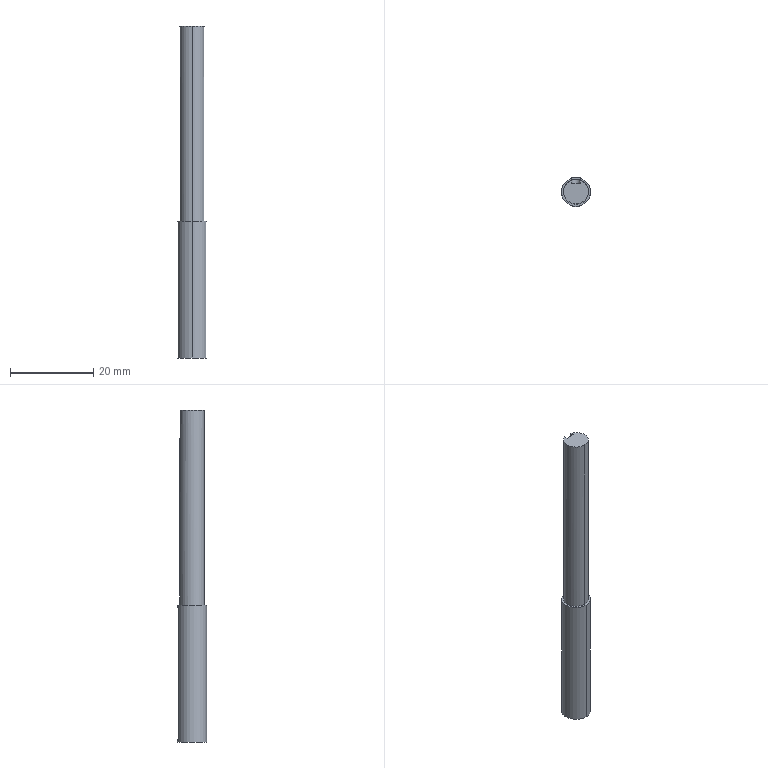Component | SolidWorks | DriveAxis-1 | 1 solid | 16 faces | box 7 x 7 x 80 mm | volume 2512 mm3 | plane 9 | cylinder 7 | commonest cylinder face diameters 6 x2 7 x2 2.5 x2 2 x1
build123d program:
from build123d import *

# Parameters (mm, degrees)
SKETCH1_R           = 3.5
BOSS_EXTRUDE1_DEPTH = 33
SKETCH2_R           = 3
BOSS_EXTRUDE2_DEPTH = 47
CUT_EXTRUDE1_DEPTH  = 1
CUT_EXTRUDE2_DEPTH  = 1


with BuildPart() as part:
    # Sketch1 → Boss-Extrude1 (new body)
    with BuildSketch(Plane(origin=(0, 0, 0), x_dir=(1, 0, 0), z_dir=(0, 1, 0))):
        with Locations(Location((0, 0, 0), (0, 0, 270))):
            Circle(SKETCH1_R)
    extrude(amount=BOSS_EXTRUDE1_DEPTH)

    # Sketch2 → Boss-Extrude2 (add)
    with BuildSketch(Plane(origin=(0, 33, 0), x_dir=(1, 0, 0), z_dir=(0, 1, 0))):
        with Locations(Location((0, 0, 0), (0, 0, 270))):
            Circle(SKETCH2_R)
    extrude(amount=BOSS_EXTRUDE2_DEPTH)

    # Sketch3 → Cut-Extrude1 (cut)
    with BuildSketch(Plane(origin=(0, 0, -3.5), x_dir=(-1, 0, 0), z_dir=(0, 0, -1))):
        with BuildLine():
            Line((1.25, 31.498), (1.25, 1.498))
            ThreePointArc((1.25, 1.498), (0, 0.2475), (-1.25, 1.498))
            Line((-1.25, 1.498), (-1.25, 31.498))
            ThreePointArc((-1.25, 31.498), (0, 32.748), (1.25, 31.498))
        make_face()
    extrude(amount=-CUT_EXTRUDE1_DEPTH, mode=Mode.SUBTRACT)

    # Sketch4 → Cut-Extrude2 (cut)
    with BuildSketch(Plane(origin=(0, 0, -3), x_dir=(-1, 0, 0), z_dir=(0, 0, -1))):
        with BuildLine():
            Line((1, 80), (1, 74))
            ThreePointArc((1, 74), (0, 73), (-1, 74))
            Line((-1, 74), (-1, 80))
            ThreePointArc((-1, 80), (0, 81), (1, 80))
        make_face()
    extrude(amount=-CUT_EXTRUDE2_DEPTH, mode=Mode.SUBTRACT)


solid = part.part

# Placed as in the assembly
solid = solid.moved(Location((48.507, -64.609, -275), (90, 0, 0)))
STEP:
#1=COLOUR_RGB('',0.7922,0.8196,0.9333);
#2=FILL_AREA_STYLE_COLOUR('',#1);
#3=FILL_AREA_STYLE('',(#2));
#4=SURFACE_STYLE_FILL_AREA(#3);
#5=SURFACE_SIDE_STYLE('',(#4));
#6=SURFACE_STYLE_USAGE(.BOTH.,#5);
#7=PRESENTATION_STYLE_ASSIGNMENT((#6));
#8=CARTESIAN_POINT('',(1.91,-2.662,-7.677));
#9=VERTEX_POINT('',#8);
#10=CARTESIAN_POINT('',(1.949,-2.432,-7.677));
#11=VERTEX_POINT('',#10);
#12=CARTESIAN_POINT('',(1.91,-2.544,-7.677));
#13=DIRECTION('',(0.,0.,1.));
#14=DIRECTION('',(0.,-1.,0.));
#15=AXIS2_PLACEMENT_3D('',#12,#13,#14);
#16=CIRCLE('',#15,0.1181);
#17=EDGE_CURVE('',#9,#11,#16,.T.);
#18=ORIENTED_EDGE('',*,*,#17,.F.);
#19=CARTESIAN_POINT('',(1.91,-2.662,-9.528));
#20=VERTEX_POINT('',#19);
#21=CARTESIAN_POINT('',(1.91,-2.662,-7.677));
#22=DIRECTION('',(0.,0.,-1.));
#23=VECTOR('',#22,39.37);
#24=LINE('',#21,#23);
#25=EDGE_CURVE('',#9,#20,#24,.T.);
#26=ORIENTED_EDGE('',*,*,#25,.T.);
#27=CARTESIAN_POINT('',(1.91,-2.426,-9.528));
#28=VERTEX_POINT('',#27);
#29=CARTESIAN_POINT('',(1.91,-2.544,-9.528));
#30=DIRECTION('',(0.,0.,1.));
#31=DIRECTION('',(0.,-1.,0.));
#32=AXIS2_PLACEMENT_3D('',#29,#30,#31);
#33=CIRCLE('',#32,0.1181);
#34=EDGE_CURVE('',#20,#28,#33,.T.);
#35=ORIENTED_EDGE('',*,*,#34,.T.);
#36=CARTESIAN_POINT('',(1.91,-2.426,-7.953));
#37=VERTEX_POINT('',#36);
#38=CARTESIAN_POINT('',(1.91,-2.426,-7.677));
#39=DIRECTION('',(0.,0.,-1.));
#40=VECTOR('',#39,39.37);
#41=LINE('',#38,#40);
#42=EDGE_CURVE('',#37,#28,#41,.T.);
#43=ORIENTED_EDGE('',*,*,#42,.F.);
#44=CARTESIAN_POINT('',(1.949,-2.432,-7.913));
#45=VERTEX_POINT('',#44);
#46=CARTESIAN_POINT('',(1.91,-2.426,-7.953));
#47=CARTESIAN_POINT('',(1.915,-2.426,-7.953));
#48=CARTESIAN_POINT('',(1.92,-2.426,-7.952));
#49=CARTESIAN_POINT('',(1.93,-2.427,-7.948));
#50=CARTESIAN_POINT('',(1.934,-2.428,-7.945));
#51=CARTESIAN_POINT('',(1.941,-2.43,-7.938));
#52=CARTESIAN_POINT('',(1.944,-2.431,-7.933));
#53=CARTESIAN_POINT('',(1.948,-2.432,-7.924));
#54=CARTESIAN_POINT('',(1.949,-2.432,-7.919));
#55=CARTESIAN_POINT('',(1.949,-2.432,-7.913));
#56=B_SPLINE_CURVE_WITH_KNOTS('',3,(#46,#47,#48,#49,#50,#51,#52,#53,#54,#55),.UNSPECIFIED.,.F.,.F.,(4,2,2,2,4),(0.001575,0.001968,0.002361,0.002755,0.003148),.UNSPECIFIED.);
#57=EDGE_CURVE('',#37,#45,#56,.T.);
#58=ORIENTED_EDGE('',*,*,#57,.T.);
#59=CARTESIAN_POINT('',(1.949,-2.432,-7.677));
#60=DIRECTION('',(0.,0.,1.));
#61=VECTOR('',#60,39.37);
#62=LINE('',#59,#61);
#63=EDGE_CURVE('',#45,#11,#62,.T.);
#64=ORIENTED_EDGE('',*,*,#63,.T.);
#65=EDGE_LOOP('',(#18,#26,#35,#43,#58,#64));
#66=FACE_OUTER_BOUND('',#65,.T.);
#67=CARTESIAN_POINT('',(1.91,-2.544,-7.677));
#68=DIRECTION('',(0.,0.,-1.));
#69=DIRECTION('',(0.,1.,0.));
#70=AXIS2_PLACEMENT_3D('',#67,#68,#69);
#71=CYLINDRICAL_SURFACE('',#70,0.1181);
#72=ADVANCED_FACE('',(#66),#71,.T.);
#73=CARTESIAN_POINT('',(1.91,-2.681,-9.528));
#74=VERTEX_POINT('',#73);
#75=CARTESIAN_POINT('',(1.91,-2.406,-9.528));
#76=VERTEX_POINT('',#75);
#77=CARTESIAN_POINT('',(1.91,-2.544,-9.528));
#78=DIRECTION('',(0.,0.,1.));
#79=DIRECTION('',(0.,-1.,0.));
#80=AXIS2_PLACEMENT_3D('',#77,#78,#79);
#81=CIRCLE('',#80,0.1378);
#82=EDGE_CURVE('',#74,#76,#81,.T.);
#83=ORIENTED_EDGE('',*,*,#82,.F.);
#84=CARTESIAN_POINT('',(1.91,-2.681,-10.827));
#85=VERTEX_POINT('',#84);
#86=CARTESIAN_POINT('',(1.91,-2.681,-9.528));
#87=DIRECTION('',(0.,0.,-1.));
#88=VECTOR('',#87,39.37);
#89=LINE('',#86,#88);
#90=EDGE_CURVE('',#74,#85,#89,.T.);
#91=ORIENTED_EDGE('',*,*,#90,.T.);
#92=CARTESIAN_POINT('',(1.91,-2.406,-10.827));
#93=VERTEX_POINT('',#92);
#94=CARTESIAN_POINT('',(1.91,-2.544,-10.827));
#95=DIRECTION('',(0.,0.,1.));
#96=DIRECTION('',(0.,-1.,0.));
#97=AXIS2_PLACEMENT_3D('',#94,#95,#96);
#98=CIRCLE('',#97,0.1378);
#99=EDGE_CURVE('',#85,#93,#98,.T.);
#100=ORIENTED_EDGE('',*,*,#99,.T.);
#101=CARTESIAN_POINT('',(1.91,-2.406,-10.817));
#102=VERTEX_POINT('',#101);
#103=CARTESIAN_POINT('',(1.91,-2.406,-9.528));
#104=DIRECTION('',(0.,0.,-1.));
#105=VECTOR('',#104,39.37);
#106=LINE('',#103,#105);
#107=EDGE_CURVE('',#102,#93,#106,.T.);
#108=ORIENTED_EDGE('',*,*,#107,.F.);
#109=CARTESIAN_POINT('',(1.959,-2.415,-10.768));
#110=VERTEX_POINT('',#109);
#111=CARTESIAN_POINT('',(1.91,-2.406,-10.817));
#112=CARTESIAN_POINT('',(1.913,-2.406,-10.817));
#113=CARTESIAN_POINT('',(1.916,-2.406,-10.817));
#114=CARTESIAN_POINT('',(1.923,-2.406,-10.815));
#115=CARTESIAN_POINT('',(1.926,-2.407,-10.814));
#116=CARTESIAN_POINT('',(1.935,-2.408,-10.811));
#117=CARTESIAN_POINT('',(1.94,-2.409,-10.807));
#118=CARTESIAN_POINT('',(1.947,-2.411,-10.8));
#119=CARTESIAN_POINT('',(1.949,-2.411,-10.798));
#120=CARTESIAN_POINT('',(1.952,-2.413,-10.793));
#121=CARTESIAN_POINT('',(1.954,-2.413,-10.79));
#122=CARTESIAN_POINT('',(1.958,-2.414,-10.781));
#123=CARTESIAN_POINT('',(1.959,-2.415,-10.774));
#124=CARTESIAN_POINT('',(1.959,-2.415,-10.768));
#125=B_SPLINE_CURVE_WITH_KNOTS('',3,(#111,#112,#113,#114,#115,#116,#117,#118,#119,#120,#121,#122,#123,#124),.UNSPECIFIED.,.F.,.F.,(4,2,2,2,2,2,4),(0.001971,0.002217,0.002463,0.002955,0.003201,0.003447,0.003939),.UNSPECIFIED.);
#126=EDGE_CURVE('',#102,#110,#125,.T.);
#127=ORIENTED_EDGE('',*,*,#126,.T.);
#128=CARTESIAN_POINT('',(1.959,-2.415,-9.587));
#129=VERTEX_POINT('',#128);
#130=CARTESIAN_POINT('',(1.959,-2.415,-9.528));
#131=DIRECTION('',(0.,0.,1.));
#132=VECTOR('',#131,39.37);
#133=LINE('',#130,#132);
#134=EDGE_CURVE('',#110,#129,#133,.T.);
#135=ORIENTED_EDGE('',*,*,#134,.T.);
#136=CARTESIAN_POINT('',(1.91,-2.406,-9.537));
#137=VERTEX_POINT('',#136);
#138=CARTESIAN_POINT('',(1.959,-2.415,-9.587));
#139=CARTESIAN_POINT('',(1.959,-2.415,-9.58));
#140=CARTESIAN_POINT('',(1.958,-2.414,-9.574));
#141=CARTESIAN_POINT('',(1.953,-2.413,-9.562));
#142=CARTESIAN_POINT('',(1.949,-2.411,-9.556));
#143=CARTESIAN_POINT('',(1.94,-2.409,-9.547));
#144=CARTESIAN_POINT('',(1.935,-2.408,-9.544));
#145=CARTESIAN_POINT('',(1.923,-2.406,-9.539));
#146=CARTESIAN_POINT('',(1.916,-2.406,-9.537));
#147=CARTESIAN_POINT('',(1.91,-2.406,-9.537));
#148=B_SPLINE_CURVE_WITH_KNOTS('',3,(#138,#139,#140,#141,#142,#143,#144,#145,#146,#147),.UNSPECIFIED.,.F.,.F.,(4,2,2,2,4),(0.,0.0004927,0.0009855,0.001478,0.001971),.UNSPECIFIED.);
#149=EDGE_CURVE('',#129,#137,#148,.T.);
#150=ORIENTED_EDGE('',*,*,#149,.T.);
#151=CARTESIAN_POINT('',(1.91,-2.406,-9.528));
#152=DIRECTION('',(0.,0.,-1.));
#153=VECTOR('',#152,39.37);
#154=LINE('',#151,#153);
#155=EDGE_CURVE('',#76,#137,#154,.T.);
#156=ORIENTED_EDGE('',*,*,#155,.F.);
#157=EDGE_LOOP('',(#83,#91,#100,#108,#127,#135,#150,#156));
#158=FACE_OUTER_BOUND('',#157,.T.);
#159=CARTESIAN_POINT('',(1.91,-2.544,-9.528));
#160=DIRECTION('',(0.,0.,-1.));
#161=DIRECTION('',(0.,1.,0.));
#162=AXIS2_PLACEMENT_3D('',#159,#160,#161);
#163=CYLINDRICAL_SURFACE('',#162,0.1378);
#164=ADVANCED_FACE('',(#158),#163,.T.);
#165=ORIENTED_EDGE('',*,*,#90,.F.);
#166=CARTESIAN_POINT('',(1.91,-2.544,-9.528));
#167=DIRECTION('',(0.,0.,1.));
#168=DIRECTION('',(0.,-1.,0.));
#169=AXIS2_PLACEMENT_3D('',#166,#167,#168);
#170=CIRCLE('',#169,0.1378);
#171=EDGE_CURVE('',#76,#74,#170,.T.);
#172=ORIENTED_EDGE('',*,*,#171,.F.);
#173=ORIENTED_EDGE('',*,*,#155,.T.);
#174=CARTESIAN_POINT('',(1.861,-2.415,-9.587));
#175=VERTEX_POINT('',#174);
#176=CARTESIAN_POINT('',(1.91,-2.406,-9.537));
#177=CARTESIAN_POINT('',(1.906,-2.406,-9.537));
#178=CARTESIAN_POINT('',(1.903,-2.406,-9.538));
#179=CARTESIAN_POINT('',(1.897,-2.406,-9.539));
#180=CARTESIAN_POINT('',(1.894,-2.407,-9.54));
#181=CARTESIAN_POINT('',(1.885,-2.408,-9.544));
#182=CARTESIAN_POINT('',(1.879,-2.409,-9.547));
#183=CARTESIAN_POINT('',(1.873,-2.411,-9.554));
#184=CARTESIAN_POINT('',(1.871,-2.411,-9.557));
#185=CARTESIAN_POINT('',(1.867,-2.413,-9.562));
#186=CARTESIAN_POINT('',(1.866,-2.413,-9.565));
#187=CARTESIAN_POINT('',(1.862,-2.414,-9.574));
#188=CARTESIAN_POINT('',(1.861,-2.415,-9.58));
#189=CARTESIAN_POINT('',(1.861,-2.415,-9.587));
#190=B_SPLINE_CURVE_WITH_KNOTS('',3,(#176,#177,#178,#179,#180,#181,#182,#183,#184,#185,#186,#187,#188,#189),.UNSPECIFIED.,.F.,.F.,(4,2,2,2,2,2,4),(0.001971,0.002217,0.002463,0.002955,0.003201,0.003447,0.003939),.UNSPECIFIED.);
#191=EDGE_CURVE('',#137,#175,#190,.T.);
#192=ORIENTED_EDGE('',*,*,#191,.T.);
#193=CARTESIAN_POINT('',(1.861,-2.415,-10.768));
#194=VERTEX_POINT('',#193);
#195=CARTESIAN_POINT('',(1.861,-2.415,-9.528));
#196=DIRECTION('',(0.,0.,-1.));
#197=VECTOR('',#196,39.37);
#198=LINE('',#195,#197);
#199=EDGE_CURVE('',#175,#194,#198,.T.);
#200=ORIENTED_EDGE('',*,*,#199,.T.);
#201=CARTESIAN_POINT('',(1.861,-2.415,-10.768));
#202=CARTESIAN_POINT('',(1.861,-2.415,-10.774));
#203=CARTESIAN_POINT('',(1.862,-2.414,-10.781));
#204=CARTESIAN_POINT('',(1.867,-2.413,-10.793));
#205=CARTESIAN_POINT('',(1.87,-2.411,-10.798));
#206=CARTESIAN_POINT('',(1.879,-2.409,-10.807));
#207=CARTESIAN_POINT('',(1.885,-2.408,-10.811));
#208=CARTESIAN_POINT('',(1.897,-2.406,-10.816));
#209=CARTESIAN_POINT('',(1.903,-2.406,-10.817));
#210=CARTESIAN_POINT('',(1.91,-2.406,-10.817));
#211=B_SPLINE_CURVE_WITH_KNOTS('',3,(#201,#202,#203,#204,#205,#206,#207,#208,#209,#210),.UNSPECIFIED.,.F.,.F.,(4,2,2,2,4),(0.,0.0004927,0.0009855,0.001478,0.001971),.UNSPECIFIED.);
#212=EDGE_CURVE('',#194,#102,#211,.T.);
#213=ORIENTED_EDGE('',*,*,#212,.T.);
#214=ORIENTED_EDGE('',*,*,#107,.T.);
#215=CARTESIAN_POINT('',(1.91,-2.544,-10.827));
#216=DIRECTION('',(0.,0.,1.));
#217=DIRECTION('',(0.,-1.,0.));
#218=AXIS2_PLACEMENT_3D('',#215,#216,#217);
#219=CIRCLE('',#218,0.1378);
#220=EDGE_CURVE('',#93,#85,#219,.T.);
#221=ORIENTED_EDGE('',*,*,#220,.T.);
#222=EDGE_LOOP('',(#165,#172,#173,#192,#200,#213,#214,#221));
#223=FACE_OUTER_BOUND('',#222,.T.);
#224=CARTESIAN_POINT('',(1.91,-2.544,-9.528));
#225=DIRECTION('',(0.,0.,-1.));
#226=DIRECTION('',(0.,1.,0.));
#227=AXIS2_PLACEMENT_3D('',#224,#225,#226);
#228=CYLINDRICAL_SURFACE('',#227,0.1378);
#229=ADVANCED_FACE('',(#223),#228,.T.);
#230=CARTESIAN_POINT('',(1.91,-2.544,-9.528));
#231=DIRECTION('',(0.,0.,1.));
#232=DIRECTION('',(0.,-1.,0.));
#233=AXIS2_PLACEMENT_3D('',#230,#231,#232);
#234=CIRCLE('',#233,0.1181);
#235=EDGE_CURVE('',#28,#20,#234,.T.);
#236=ORIENTED_EDGE('',*,*,#235,.F.);
#237=ORIENTED_EDGE('',*,*,#34,.F.);
#238=EDGE_LOOP('',(#236,#237));
#239=FACE_BOUND('',#238,.T.);
#240=ORIENTED_EDGE('',*,*,#171,.T.);
#241=ORIENTED_EDGE('',*,*,#82,.T.);
#242=EDGE_LOOP('',(#240,#241));
#243=FACE_OUTER_BOUND('',#242,.T.);
#244=CARTESIAN_POINT('',(1.91,-2.544,-9.528));
#245=DIRECTION('',(0.,0.,1.));
#246=DIRECTION('',(0.,-1.,0.));
#247=AXIS2_PLACEMENT_3D('',#244,#245,#246);
#248=PLANE('',#247);
#249=ADVANCED_FACE('',(#239,#243),#248,.T.);
#250=ORIENTED_EDGE('',*,*,#220,.F.);
#251=ORIENTED_EDGE('',*,*,#99,.F.);
#252=EDGE_LOOP('',(#250,#251));
#253=FACE_OUTER_BOUND('',#252,.T.);
#254=CARTESIAN_POINT('',(1.91,-2.544,-10.827));
#255=DIRECTION('',(0.,0.,1.));
#256=DIRECTION('',(0.,-1.,0.));
#257=AXIS2_PLACEMENT_3D('',#254,#255,#256);
#258=PLANE('',#257);
#259=ADVANCED_FACE('',(#253),#258,.F.);
#260=ORIENTED_EDGE('',*,*,#25,.F.);
#261=CARTESIAN_POINT('',(1.87,-2.432,-7.677));
#262=VERTEX_POINT('',#261);
#263=CARTESIAN_POINT('',(1.91,-2.544,-7.677));
#264=DIRECTION('',(0.,0.,1.));
#265=DIRECTION('',(0.,-1.,0.));
#266=AXIS2_PLACEMENT_3D('',#263,#264,#265);
#267=CIRCLE('',#266,0.1181);
#268=EDGE_CURVE('',#262,#9,#267,.T.);
#269=ORIENTED_EDGE('',*,*,#268,.F.);
#270=CARTESIAN_POINT('',(1.87,-2.432,-7.913));
#271=VERTEX_POINT('',#270);
#272=CARTESIAN_POINT('',(1.87,-2.432,-7.677));
#273=DIRECTION('',(0.,0.,-1.));
#274=VECTOR('',#273,39.37);
#275=LINE('',#272,#274);
#276=EDGE_CURVE('',#262,#271,#275,.T.);
#277=ORIENTED_EDGE('',*,*,#276,.T.);
#278=CARTESIAN_POINT('',(1.87,-2.432,-7.913));
#279=CARTESIAN_POINT('',(1.87,-2.432,-7.919));
#280=CARTESIAN_POINT('',(1.871,-2.432,-7.924));
#281=CARTESIAN_POINT('',(1.875,-2.431,-7.933));
#282=CARTESIAN_POINT('',(1.878,-2.43,-7.938));
#283=CARTESIAN_POINT('',(1.885,-2.428,-7.945));
#284=CARTESIAN_POINT('',(1.89,-2.427,-7.948));
#285=CARTESIAN_POINT('',(1.899,-2.426,-7.952));
#286=CARTESIAN_POINT('',(1.905,-2.426,-7.953));
#287=CARTESIAN_POINT('',(1.91,-2.426,-7.953));
#288=B_SPLINE_CURVE_WITH_KNOTS('',3,(#278,#279,#280,#281,#282,#283,#284,#285,#286,#287),.UNSPECIFIED.,.F.,.F.,(4,2,2,2,4),(0.,0.0003937,0.0007875,0.001181,0.001575),.UNSPECIFIED.);
#289=EDGE_CURVE('',#271,#37,#288,.T.);
#290=ORIENTED_EDGE('',*,*,#289,.T.);
#291=ORIENTED_EDGE('',*,*,#42,.T.);
#292=ORIENTED_EDGE('',*,*,#235,.T.);
#293=EDGE_LOOP('',(#260,#269,#277,#290,#291,#292));
#294=FACE_OUTER_BOUND('',#293,.T.);
#295=CARTESIAN_POINT('',(1.91,-2.544,-7.677));
#296=DIRECTION('',(0.,0.,-1.));
#297=DIRECTION('',(0.,1.,0.));
#298=AXIS2_PLACEMENT_3D('',#295,#296,#297);
#299=CYLINDRICAL_SURFACE('',#298,0.1181);
#300=ADVANCED_FACE('',(#294),#299,.T.);
#301=CARTESIAN_POINT('',(1.87,-2.465,-7.677));
#302=VERTEX_POINT('',#301);
#303=CARTESIAN_POINT('',(1.87,-2.465,-7.677));
#304=DIRECTION('',(0.,1.,0.));
#305=VECTOR('',#304,39.37);
#306=LINE('',#303,#305);
#307=EDGE_CURVE('',#302,#262,#306,.T.);
#308=ORIENTED_EDGE('',*,*,#307,.T.);
#309=ORIENTED_EDGE('',*,*,#268,.T.);
#310=ORIENTED_EDGE('',*,*,#17,.T.);
#311=CARTESIAN_POINT('',(1.949,-2.465,-7.677));
#312=VERTEX_POINT('',#311);
#313=CARTESIAN_POINT('',(1.949,-2.465,-7.677));
#314=DIRECTION('',(0.,1.,0.));
#315=VECTOR('',#314,39.37);
#316=LINE('',#313,#315);
#317=EDGE_CURVE('',#312,#11,#316,.T.);
#318=ORIENTED_EDGE('',*,*,#317,.F.);
#319=CARTESIAN_POINT('',(1.91,-2.465,-7.677));
#320=DIRECTION('',(-1.,0.,0.));
#321=VECTOR('',#320,39.37);
#322=LINE('',#319,#321);
#323=EDGE_CURVE('',#312,#302,#322,.T.);
#324=ORIENTED_EDGE('',*,*,#323,.T.);
#325=EDGE_LOOP('',(#308,#309,#310,#318,#324));
#326=FACE_OUTER_BOUND('',#325,.T.);
#327=CARTESIAN_POINT('',(1.91,-2.544,-7.677));
#328=DIRECTION('',(0.,0.,1.));
#329=DIRECTION('',(0.,-1.,0.));
#330=AXIS2_PLACEMENT_3D('',#327,#328,#329);
#331=PLANE('',#330);
#332=ADVANCED_FACE('',(#326),#331,.T.);
#333=CARTESIAN_POINT('',(1.959,-2.445,-9.587));
#334=VERTEX_POINT('',#333);
#335=CARTESIAN_POINT('',(1.959,-2.445,-9.587));
#336=DIRECTION('',(0.,1.,0.));
#337=VECTOR('',#336,39.37);
#338=LINE('',#335,#337);
#339=EDGE_CURVE('',#334,#129,#338,.T.);
#340=ORIENTED_EDGE('',*,*,#339,.F.);
#341=CARTESIAN_POINT('',(1.861,-2.445,-9.587));
#342=VERTEX_POINT('',#341);
#343=CARTESIAN_POINT('',(1.91,-2.445,-9.587));
#344=DIRECTION('',(0.,1.,0.));
#345=DIRECTION('',(-1.,0.,0.));
#346=AXIS2_PLACEMENT_3D('',#343,#344,#345);
#347=CIRCLE('',#346,0.04921);
#348=EDGE_CURVE('',#342,#334,#347,.T.);
#349=ORIENTED_EDGE('',*,*,#348,.F.);
#350=CARTESIAN_POINT('',(1.861,-2.445,-9.587));
#351=DIRECTION('',(0.,1.,0.));
#352=VECTOR('',#351,39.37);
#353=LINE('',#350,#352);
#354=EDGE_CURVE('',#342,#175,#353,.T.);
#355=ORIENTED_EDGE('',*,*,#354,.T.);
#356=ORIENTED_EDGE('',*,*,#191,.F.);
#357=ORIENTED_EDGE('',*,*,#149,.F.);
#358=EDGE_LOOP('',(#340,#349,#355,#356,#357));
#359=FACE_OUTER_BOUND('',#358,.T.);
#360=CARTESIAN_POINT('',(1.91,-2.445,-9.587));
#361=DIRECTION('',(0.,1.,0.));
#362=DIRECTION('',(-1.,0.,0.));
#363=AXIS2_PLACEMENT_3D('',#360,#361,#362);
#364=CYLINDRICAL_SURFACE('',#363,0.04921);
#365=ADVANCED_FACE('',(#359),#364,.F.);
#366=ORIENTED_EDGE('',*,*,#354,.F.);
#367=CARTESIAN_POINT('',(1.861,-2.445,-10.768));
#368=VERTEX_POINT('',#367);
#369=CARTESIAN_POINT('',(1.861,-2.445,-9.587));
#370=DIRECTION('',(-0.,0.,1.));
#371=VECTOR('',#370,39.37);
#372=LINE('',#369,#371);
#373=EDGE_CURVE('',#368,#342,#372,.T.);
#374=ORIENTED_EDGE('',*,*,#373,.F.);
#375=CARTESIAN_POINT('',(1.861,-2.445,-10.768));
#376=DIRECTION('',(0.,1.,0.));
#377=VECTOR('',#376,39.37);
#378=LINE('',#375,#377);
#379=EDGE_CURVE('',#368,#194,#378,.T.);
#380=ORIENTED_EDGE('',*,*,#379,.T.);
#381=ORIENTED_EDGE('',*,*,#199,.F.);
#382=EDGE_LOOP('',(#366,#374,#380,#381));
#383=FACE_OUTER_BOUND('',#382,.T.);
#384=CARTESIAN_POINT('',(1.861,-2.445,-9.587));
#385=DIRECTION('',(-1.,0.,-0.));
#386=DIRECTION('',(0.,0.,-1.));
#387=AXIS2_PLACEMENT_3D('',#384,#385,#386);
#388=PLANE('',#387);
#389=ADVANCED_FACE('',(#383),#388,.F.);
#390=ORIENTED_EDGE('',*,*,#379,.F.);
#391=CARTESIAN_POINT('',(1.959,-2.445,-10.768));
#392=VERTEX_POINT('',#391);
#393=CARTESIAN_POINT('',(1.91,-2.445,-10.768));
#394=DIRECTION('',(0.,1.,0.));
#395=DIRECTION('',(-1.,0.,0.));
#396=AXIS2_PLACEMENT_3D('',#393,#394,#395);
#397=CIRCLE('',#396,0.04921);
#398=EDGE_CURVE('',#392,#368,#397,.T.);
#399=ORIENTED_EDGE('',*,*,#398,.F.);
#400=CARTESIAN_POINT('',(1.959,-2.445,-10.768));
#401=DIRECTION('',(0.,1.,0.));
#402=VECTOR('',#401,39.37);
#403=LINE('',#400,#402);
#404=EDGE_CURVE('',#392,#110,#403,.T.);
#405=ORIENTED_EDGE('',*,*,#404,.T.);
#406=ORIENTED_EDGE('',*,*,#126,.F.);
#407=ORIENTED_EDGE('',*,*,#212,.F.);
#408=EDGE_LOOP('',(#390,#399,#405,#406,#407));
#409=FACE_OUTER_BOUND('',#408,.T.);
#410=CARTESIAN_POINT('',(1.91,-2.445,-10.768));
#411=DIRECTION('',(0.,1.,0.));
#412=DIRECTION('',(-1.,0.,0.));
#413=AXIS2_PLACEMENT_3D('',#410,#411,#412);
#414=CYLINDRICAL_SURFACE('',#413,0.04921);
#415=ADVANCED_FACE('',(#409),#414,.F.);
#416=ORIENTED_EDGE('',*,*,#404,.F.);
#417=CARTESIAN_POINT('',(1.959,-2.445,-9.587));
#418=DIRECTION('',(-0.,0.,-1.));
#419=VECTOR('',#418,39.37);
#420=LINE('',#417,#419);
#421=EDGE_CURVE('',#334,#392,#420,.T.);
#422=ORIENTED_EDGE('',*,*,#421,.F.);
#423=ORIENTED_EDGE('',*,*,#339,.T.);
#424=ORIENTED_EDGE('',*,*,#134,.F.);
#425=EDGE_LOOP('',(#416,#422,#423,#424));
#426=FACE_OUTER_BOUND('',#425,.T.);
#427=CARTESIAN_POINT('',(1.959,-2.445,-9.587));
#428=DIRECTION('',(1.,0.,-0.));
#429=DIRECTION('',(0.,0.,1.));
#430=AXIS2_PLACEMENT_3D('',#427,#428,#429);
#431=PLANE('',#430);
#432=ADVANCED_FACE('',(#426),#431,.F.);
#433=ORIENTED_EDGE('',*,*,#348,.T.);
#434=ORIENTED_EDGE('',*,*,#421,.T.);
#435=ORIENTED_EDGE('',*,*,#398,.T.);
#436=ORIENTED_EDGE('',*,*,#373,.T.);
#437=EDGE_LOOP('',(#433,#434,#435,#436));
#438=FACE_OUTER_BOUND('',#437,.T.);
#439=CARTESIAN_POINT('',(1.91,-2.445,-9.587));
#440=DIRECTION('',(0.,1.,0.));
#441=DIRECTION('',(-1.,0.,0.));
#442=AXIS2_PLACEMENT_3D('',#439,#440,#441);
#443=PLANE('',#442);
#444=ADVANCED_FACE('',(#438),#443,.T.);
#445=CARTESIAN_POINT('',(1.87,-2.465,-7.913));
#446=VERTEX_POINT('',#445);
#447=CARTESIAN_POINT('',(1.87,-2.465,-7.913));
#448=DIRECTION('',(0.,1.,0.));
#449=VECTOR('',#448,39.37);
#450=LINE('',#447,#449);
#451=EDGE_CURVE('',#446,#271,#450,.T.);
#452=ORIENTED_EDGE('',*,*,#451,.F.);
#453=CARTESIAN_POINT('',(1.949,-2.465,-7.913));
#454=VERTEX_POINT('',#453);
#455=CARTESIAN_POINT('',(1.91,-2.465,-7.913));
#456=DIRECTION('',(0.,1.,0.));
#457=DIRECTION('',(-1.,0.,0.));
#458=AXIS2_PLACEMENT_3D('',#455,#456,#457);
#459=CIRCLE('',#458,0.03937);
#460=EDGE_CURVE('',#454,#446,#459,.T.);
#461=ORIENTED_EDGE('',*,*,#460,.F.);
#462=CARTESIAN_POINT('',(1.949,-2.465,-7.913));
#463=DIRECTION('',(0.,1.,0.));
#464=VECTOR('',#463,39.37);
#465=LINE('',#462,#464);
#466=EDGE_CURVE('',#454,#45,#465,.T.);
#467=ORIENTED_EDGE('',*,*,#466,.T.);
#468=ORIENTED_EDGE('',*,*,#57,.F.);
#469=ORIENTED_EDGE('',*,*,#289,.F.);
#470=EDGE_LOOP('',(#452,#461,#467,#468,#469));
#471=FACE_OUTER_BOUND('',#470,.T.);
#472=CARTESIAN_POINT('',(1.91,-2.465,-7.913));
#473=DIRECTION('',(0.,1.,0.));
#474=DIRECTION('',(-1.,0.,0.));
#475=AXIS2_PLACEMENT_3D('',#472,#473,#474);
#476=CYLINDRICAL_SURFACE('',#475,0.03937);
#477=ADVANCED_FACE('',(#471),#476,.F.);
#478=ORIENTED_EDGE('',*,*,#307,.F.);
#479=CARTESIAN_POINT('',(1.87,-2.465,-7.677));
#480=DIRECTION('',(0.,0.,1.));
#481=VECTOR('',#480,39.37);
#482=LINE('',#479,#481);
#483=EDGE_CURVE('',#446,#302,#482,.T.);
#484=ORIENTED_EDGE('',*,*,#483,.F.);
#485=ORIENTED_EDGE('',*,*,#451,.T.);
#486=ORIENTED_EDGE('',*,*,#276,.F.);
#487=EDGE_LOOP('',(#478,#484,#485,#486));
#488=FACE_OUTER_BOUND('',#487,.T.);
#489=CARTESIAN_POINT('',(1.87,-2.465,-7.677));
#490=DIRECTION('',(-1.,0.,0.));
#491=DIRECTION('',(0.,-1.,0.));
#492=AXIS2_PLACEMENT_3D('',#489,#490,#491);
#493=PLANE('',#492);
#494=ADVANCED_FACE('',(#488),#493,.F.);
#495=ORIENTED_EDGE('',*,*,#466,.F.);
#496=CARTESIAN_POINT('',(1.949,-2.465,-7.677));
#497=DIRECTION('',(0.,0.,-1.));
#498=VECTOR('',#497,39.37);
#499=LINE('',#496,#498);
#500=EDGE_CURVE('',#312,#454,#499,.T.);
#501=ORIENTED_EDGE('',*,*,#500,.F.);
#502=ORIENTED_EDGE('',*,*,#317,.T.);
#503=ORIENTED_EDGE('',*,*,#63,.F.);
#504=EDGE_LOOP('',(#495,#501,#502,#503));
#505=FACE_OUTER_BOUND('',#504,.T.);
#506=CARTESIAN_POINT('',(1.949,-2.465,-7.677));
#507=DIRECTION('',(1.,0.,0.));
#508=DIRECTION('',(0.,1.,0.));
#509=AXIS2_PLACEMENT_3D('',#506,#507,#508);
#510=PLANE('',#509);
#511=ADVANCED_FACE('',(#505),#510,.F.);
#512=ORIENTED_EDGE('',*,*,#500,.T.);
#513=ORIENTED_EDGE('',*,*,#460,.T.);
#514=ORIENTED_EDGE('',*,*,#483,.T.);
#515=ORIENTED_EDGE('',*,*,#323,.F.);
#516=EDGE_LOOP('',(#512,#513,#514,#515));
#517=FACE_OUTER_BOUND('',#516,.T.);
#518=CARTESIAN_POINT('',(1.91,-2.465,-7.677));
#519=DIRECTION('',(0.,1.,0.));
#520=DIRECTION('',(-1.,0.,0.));
#521=AXIS2_PLACEMENT_3D('',#518,#519,#520);
#522=PLANE('',#521);
#523=ADVANCED_FACE('',(#517),#522,.T.);
#524=CLOSED_SHELL('',(#72,#164,#229,#249,#259,#300,#332,#365,#389,#415,#432,#444,#477,#494,#511,#523));
#525=MANIFOLD_SOLID_BREP('',#524);
#526=STYLED_ITEM('',(#7),#525);
#527=PRESENTATION_LAYER_ASSIGNMENT('','',(#526));
#528=CARTESIAN_POINT('',(0.,0.,0.));
#529=DIRECTION('',(0.,0.,1.));
#530=DIRECTION('',(1.,0.,0.));
#531=AXIS2_PLACEMENT_3D('',#528,#529,#530);
#532=(LENGTH_UNIT()NAMED_UNIT(*)SI_UNIT($,.METRE.));
#533=LENGTH_MEASURE_WITH_UNIT(LENGTH_MEASURE(0.0254),#532);
#534=DIMENSIONAL_EXPONENTS(1.,0.,0.,0.,0.,0.,0.);
#535=(CONVERSION_BASED_UNIT('',#533)LENGTH_UNIT()NAMED_UNIT(#534));
#536=UNCERTAINTY_MEASURE_WITH_UNIT(LENGTH_MEASURE(0.00001),#535,'','');
#537=(NAMED_UNIT(*)PLANE_ANGLE_UNIT()SI_UNIT($,.RADIAN.));
#538=(NAMED_UNIT(*)SI_UNIT($,.STERADIAN.)SOLID_ANGLE_UNIT());
#539=(GEOMETRIC_REPRESENTATION_CONTEXT(3)GLOBAL_UNCERTAINTY_ASSIGNED_CONTEXT((#536))GLOBAL_UNIT_ASSIGNED_CONTEXT((#535,#537,#538))REPRESENTATION_CONTEXT('',''));
#540=ADVANCED_BREP_SHAPE_REPRESENTATION('',(#525,#531),#539);
#541=(LENGTH_UNIT()NAMED_UNIT(*)SI_UNIT($,.METRE.));
#542=LENGTH_MEASURE_WITH_UNIT(LENGTH_MEASURE(0.0254),#541);
#543=DIMENSIONAL_EXPONENTS(1.,0.,0.,0.,0.,0.,0.);
#544=(CONVERSION_BASED_UNIT('',#542)LENGTH_UNIT()NAMED_UNIT(#543));
#545=UNCERTAINTY_MEASURE_WITH_UNIT(LENGTH_MEASURE(0.00001),#544,'','');
#546=(NAMED_UNIT(*)PLANE_ANGLE_UNIT()SI_UNIT($,.RADIAN.));
#547=(NAMED_UNIT(*)SI_UNIT($,.STERADIAN.)SOLID_ANGLE_UNIT());
#548=(GEOMETRIC_REPRESENTATION_CONTEXT(3)GLOBAL_UNCERTAINTY_ASSIGNED_CONTEXT((#545))GLOBAL_UNIT_ASSIGNED_CONTEXT((#544,#546,#547))REPRESENTATION_CONTEXT('',''));
#549=MECHANICAL_DESIGN_GEOMETRIC_PRESENTATION_REPRESENTATION('',(#526),#548);